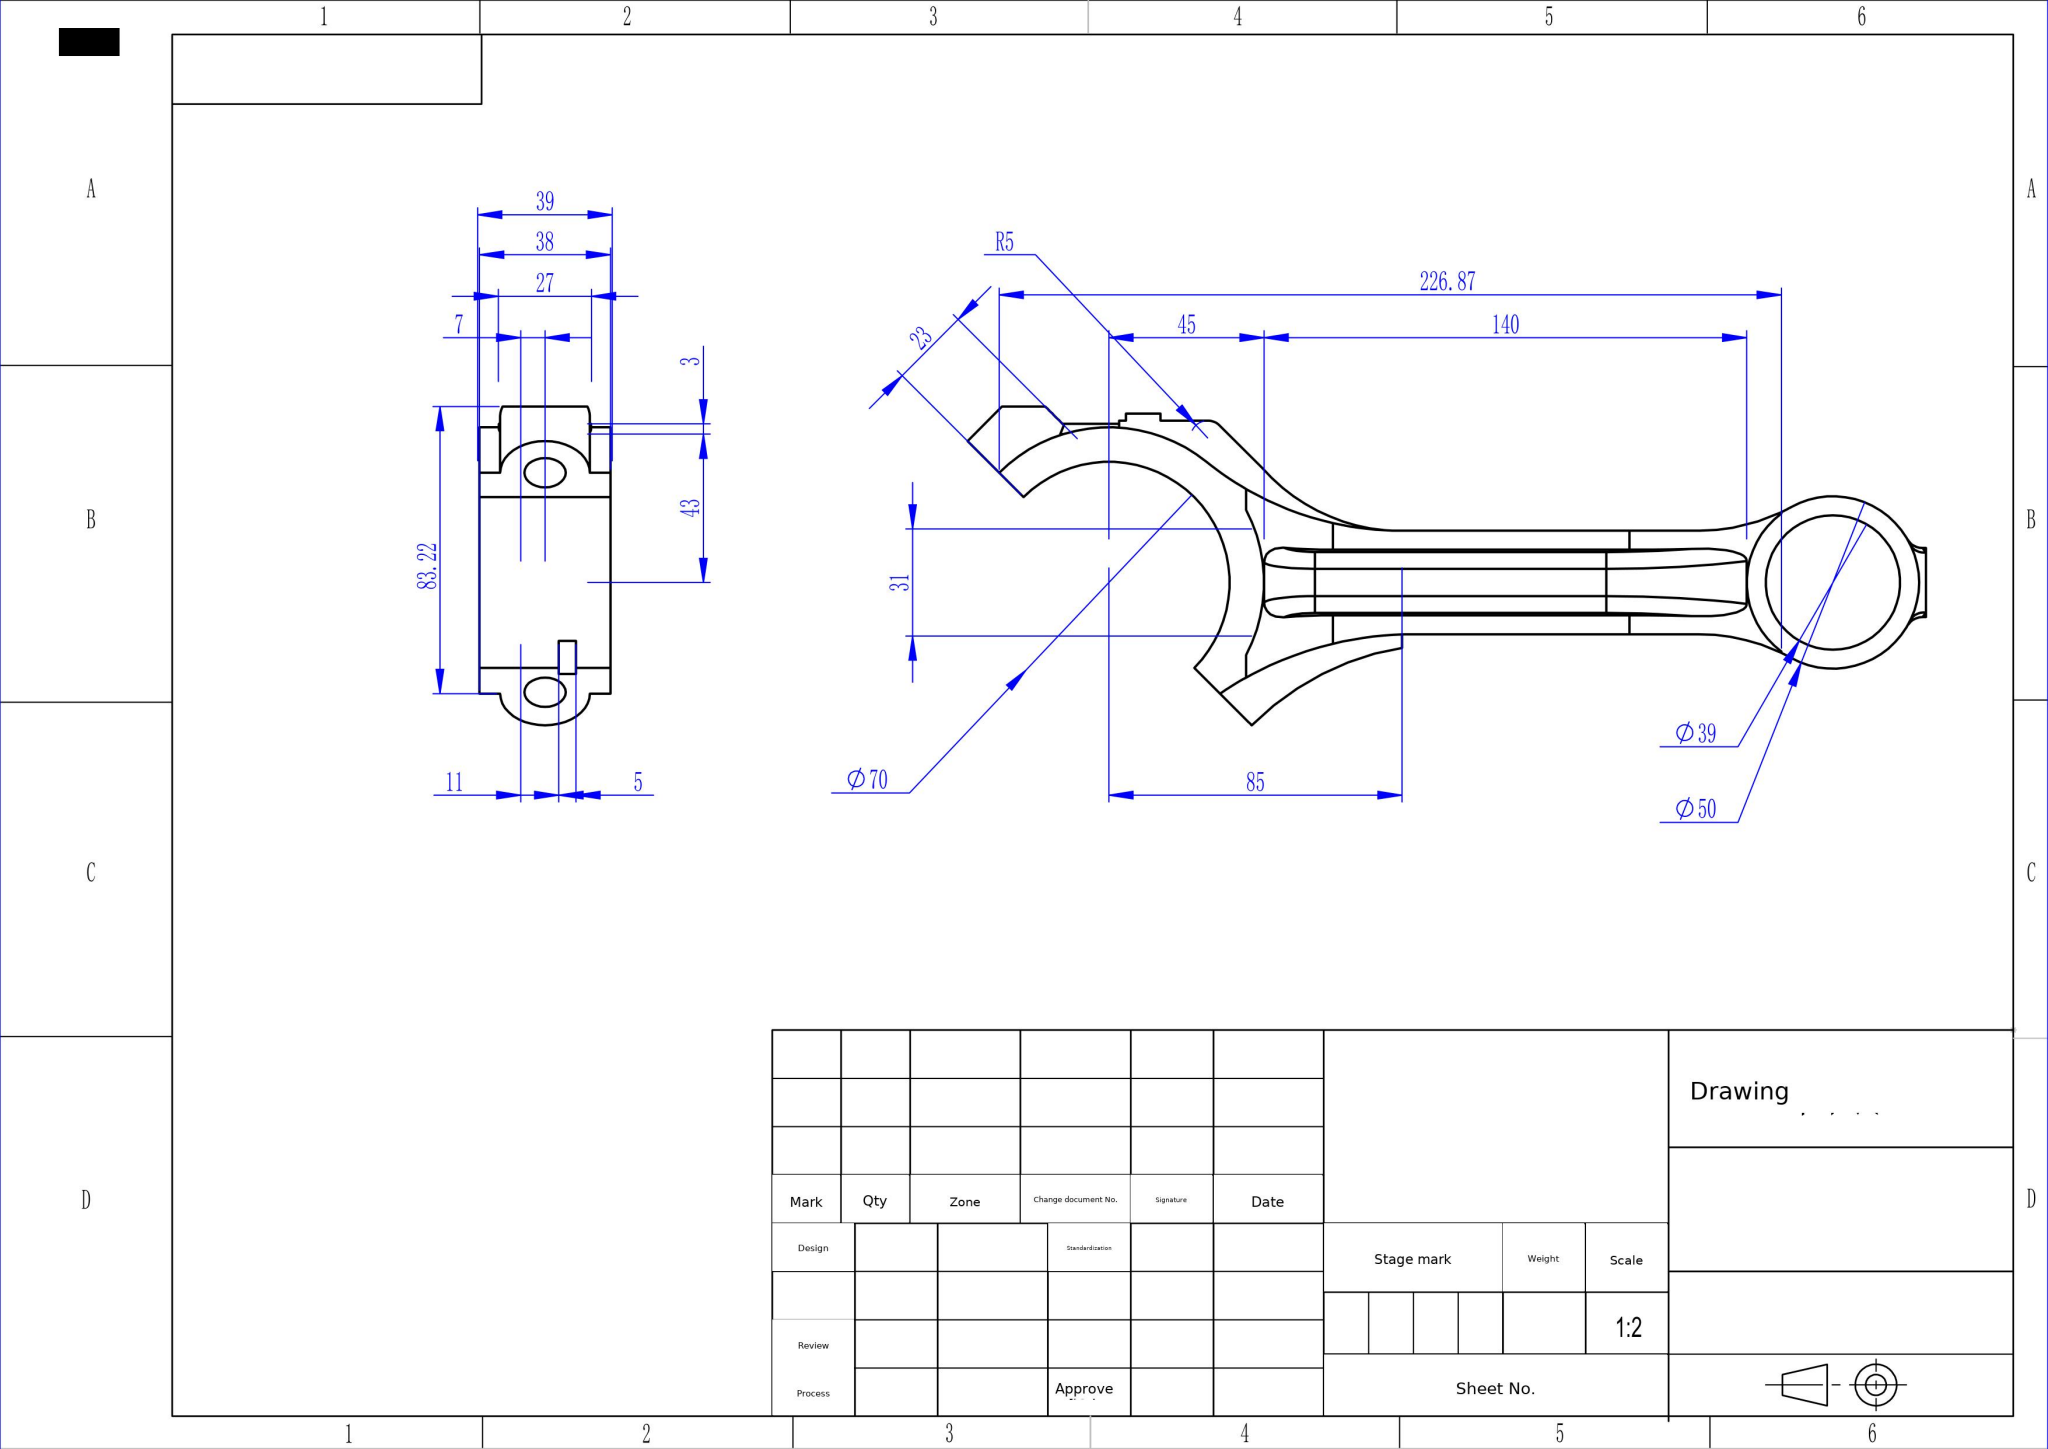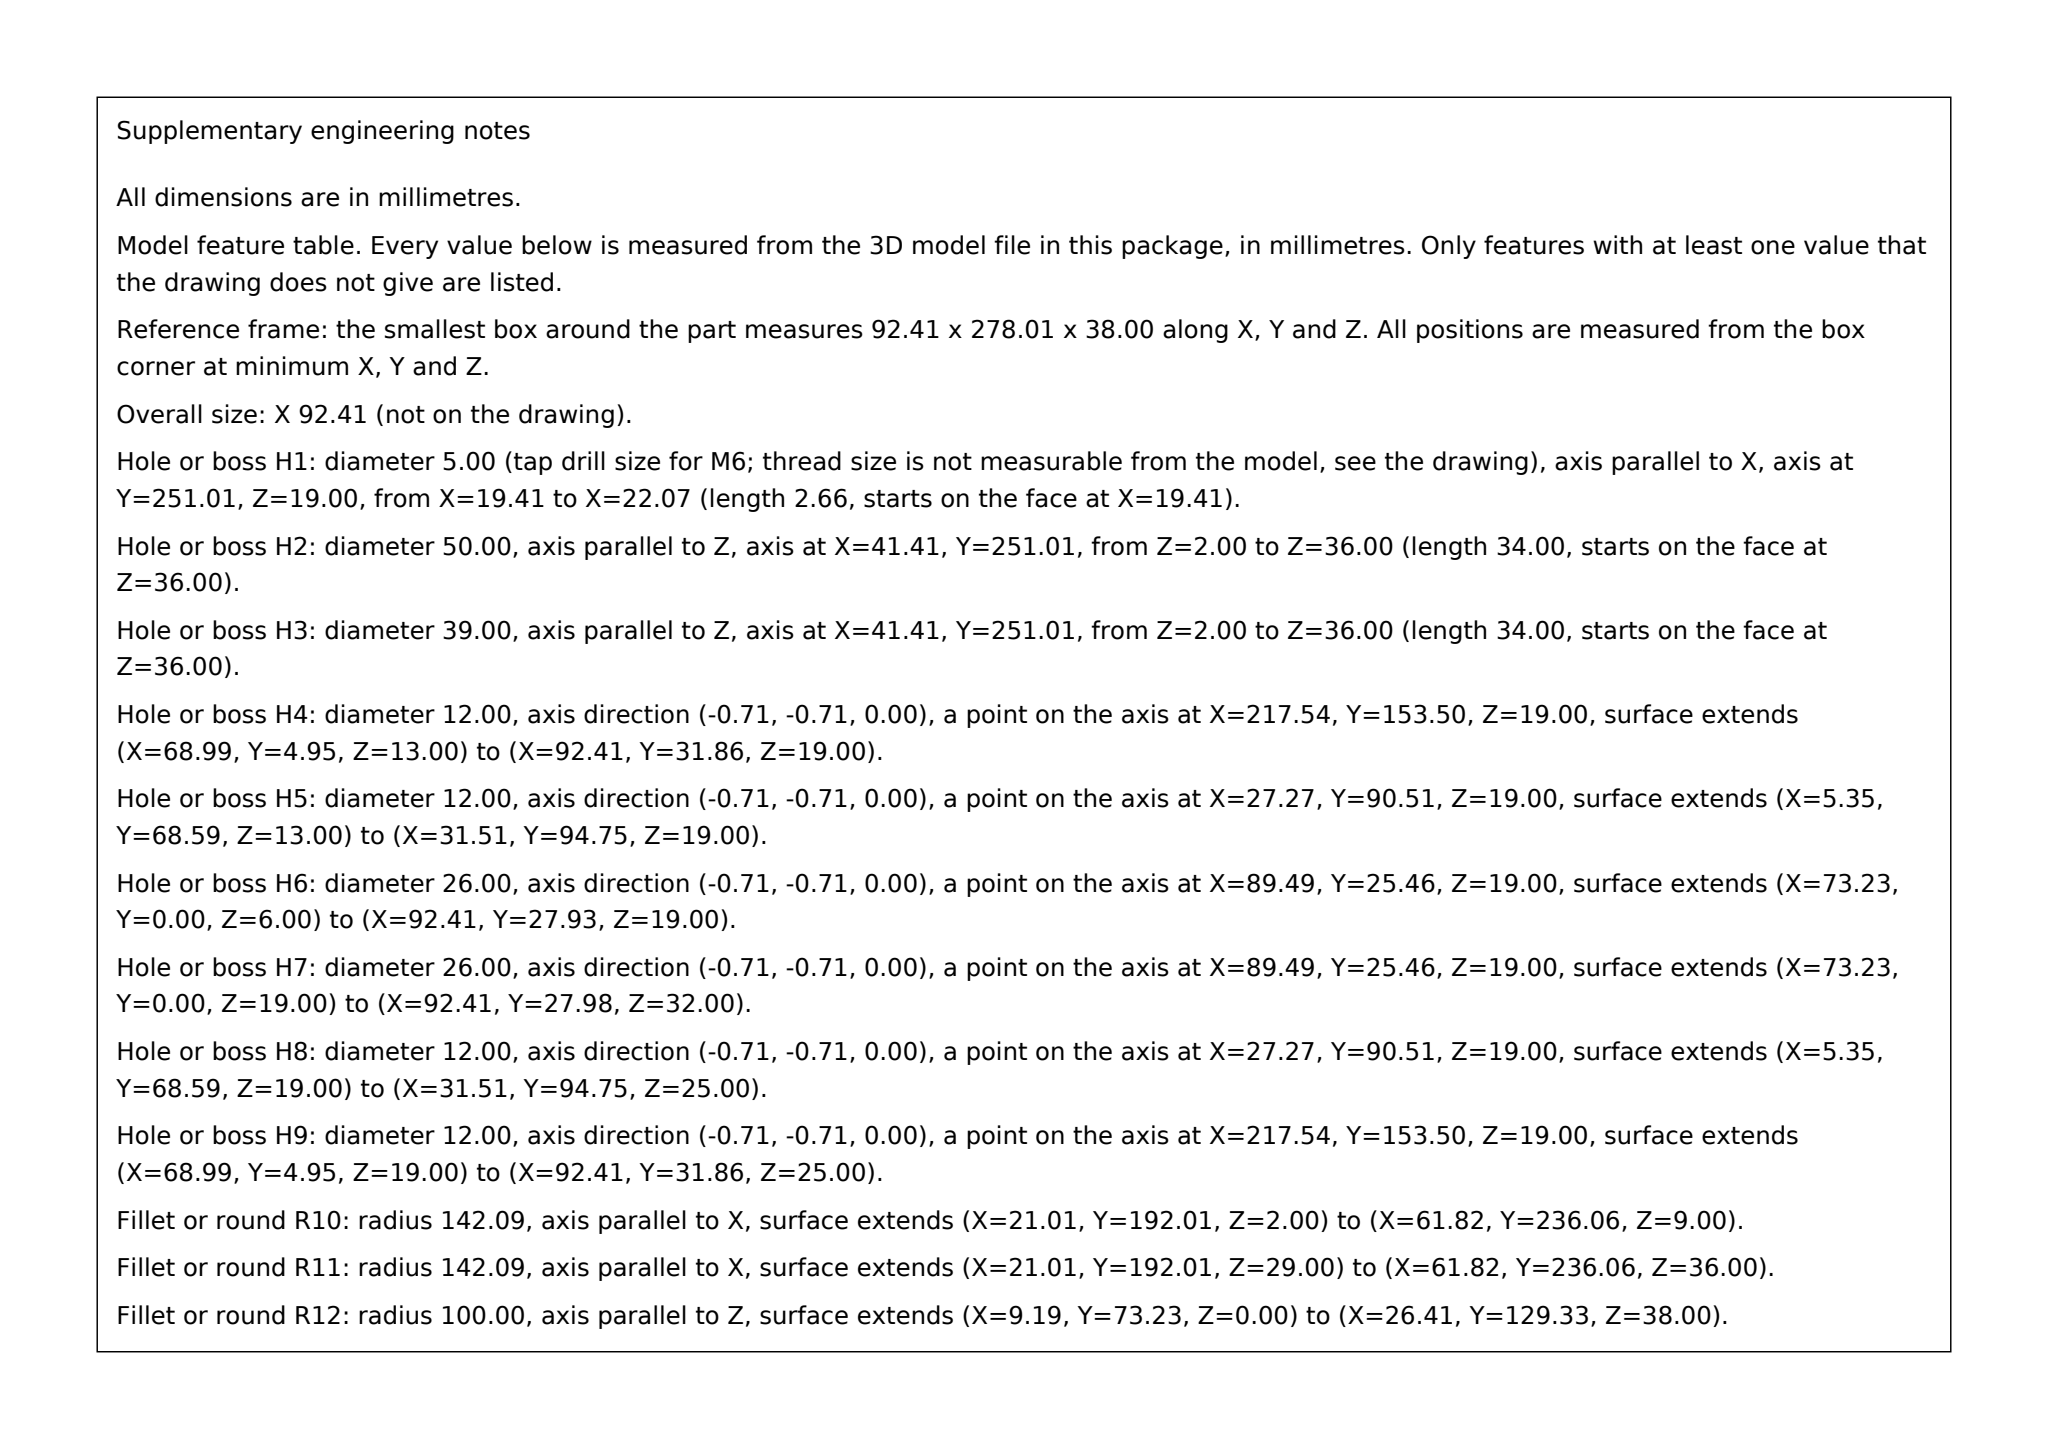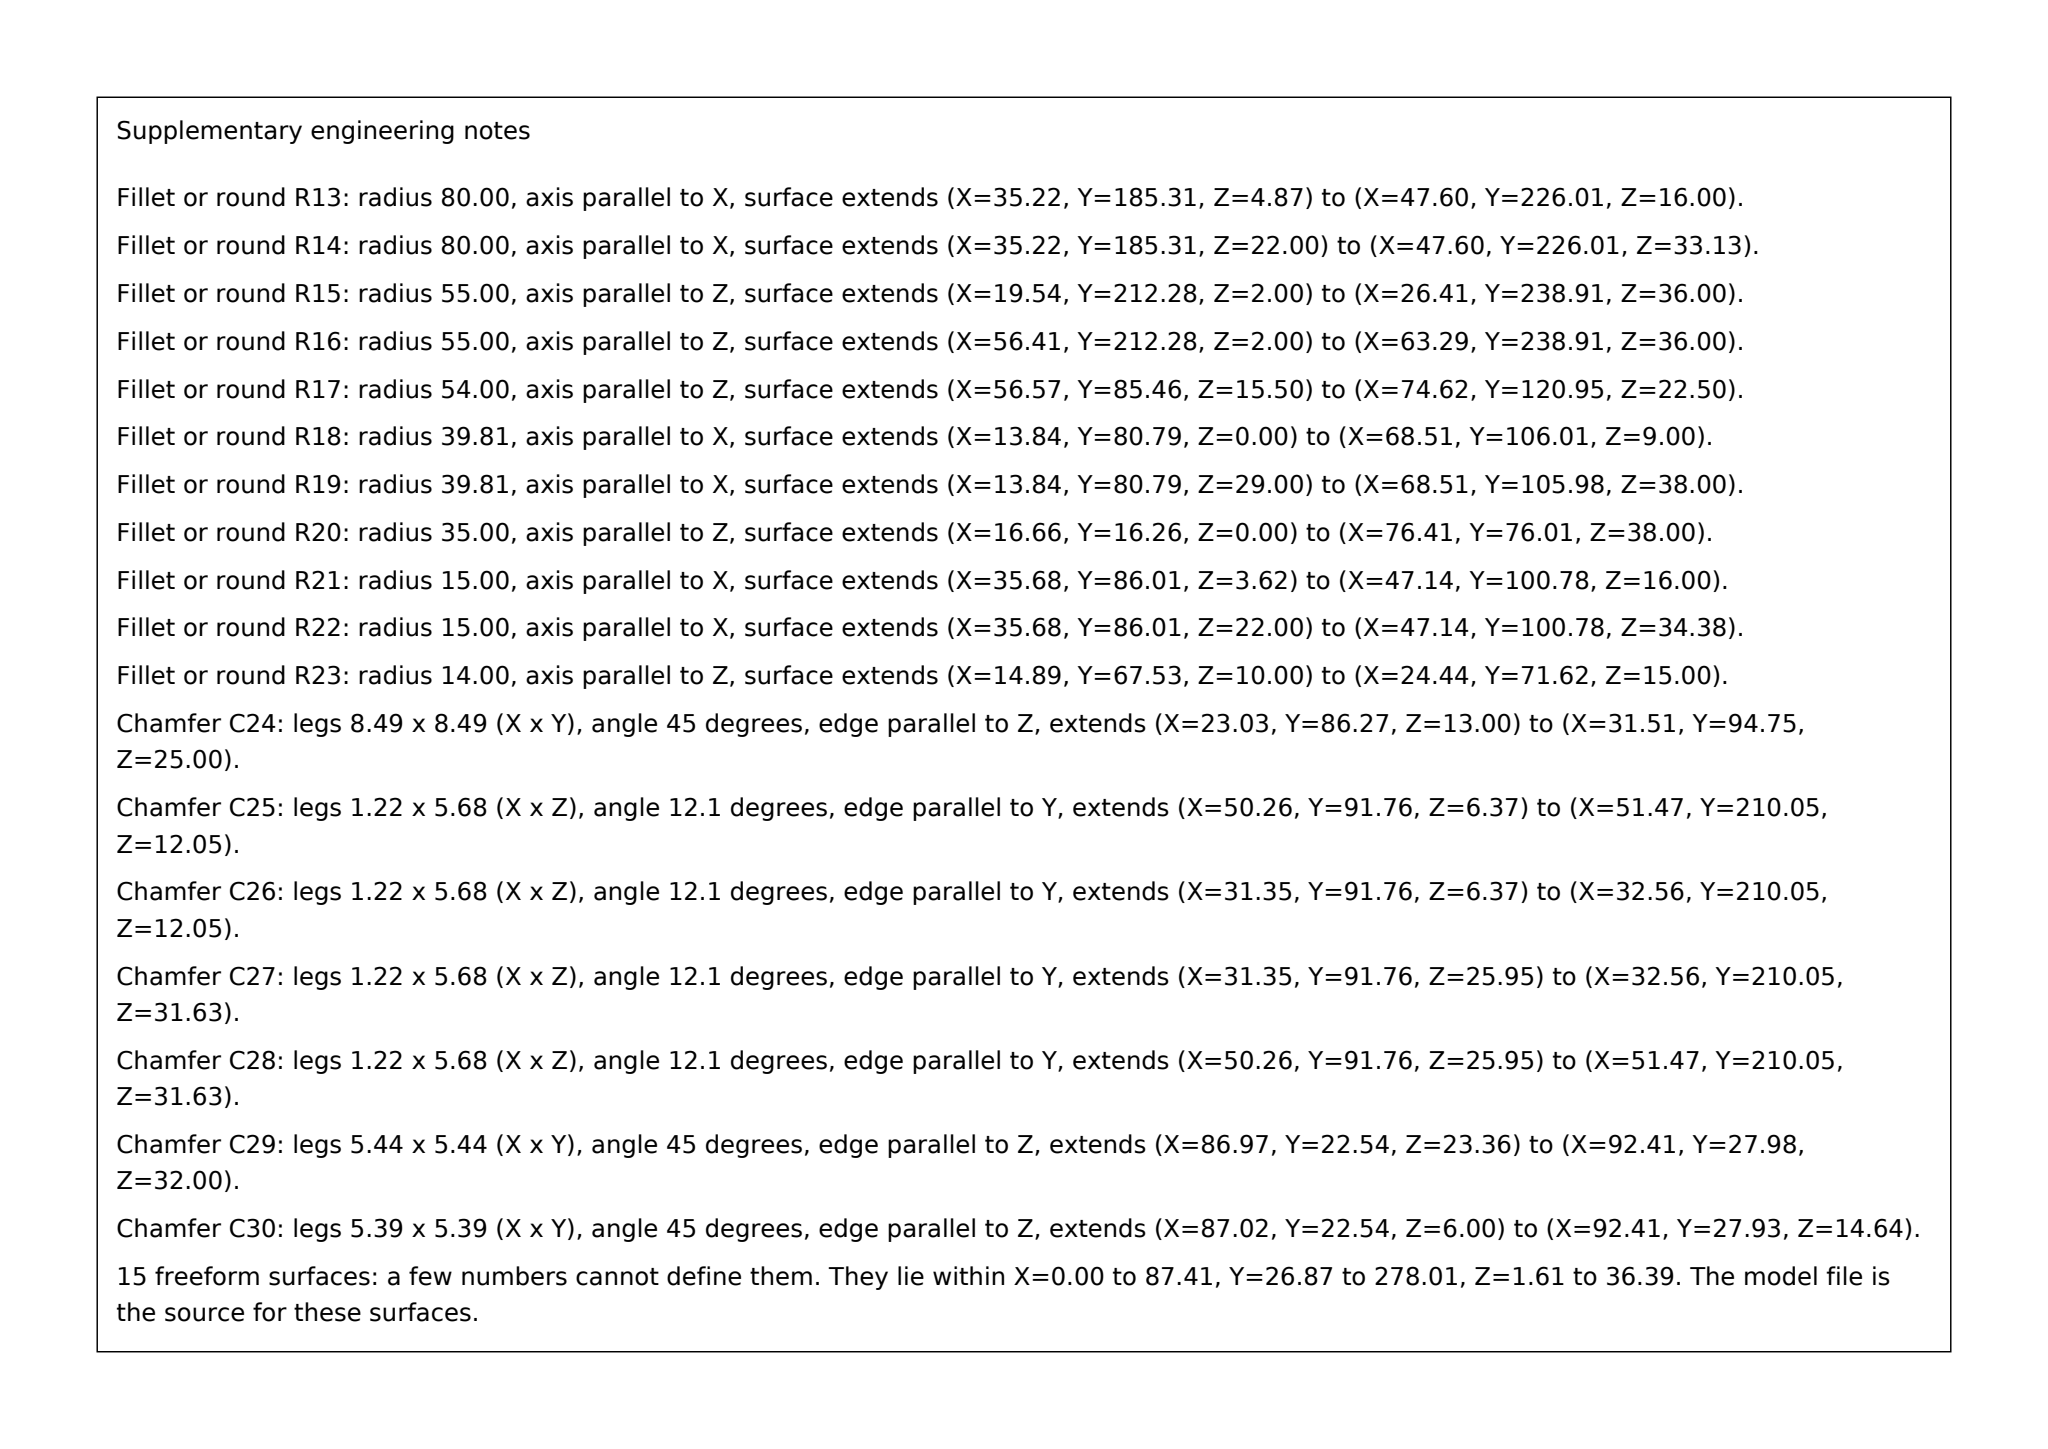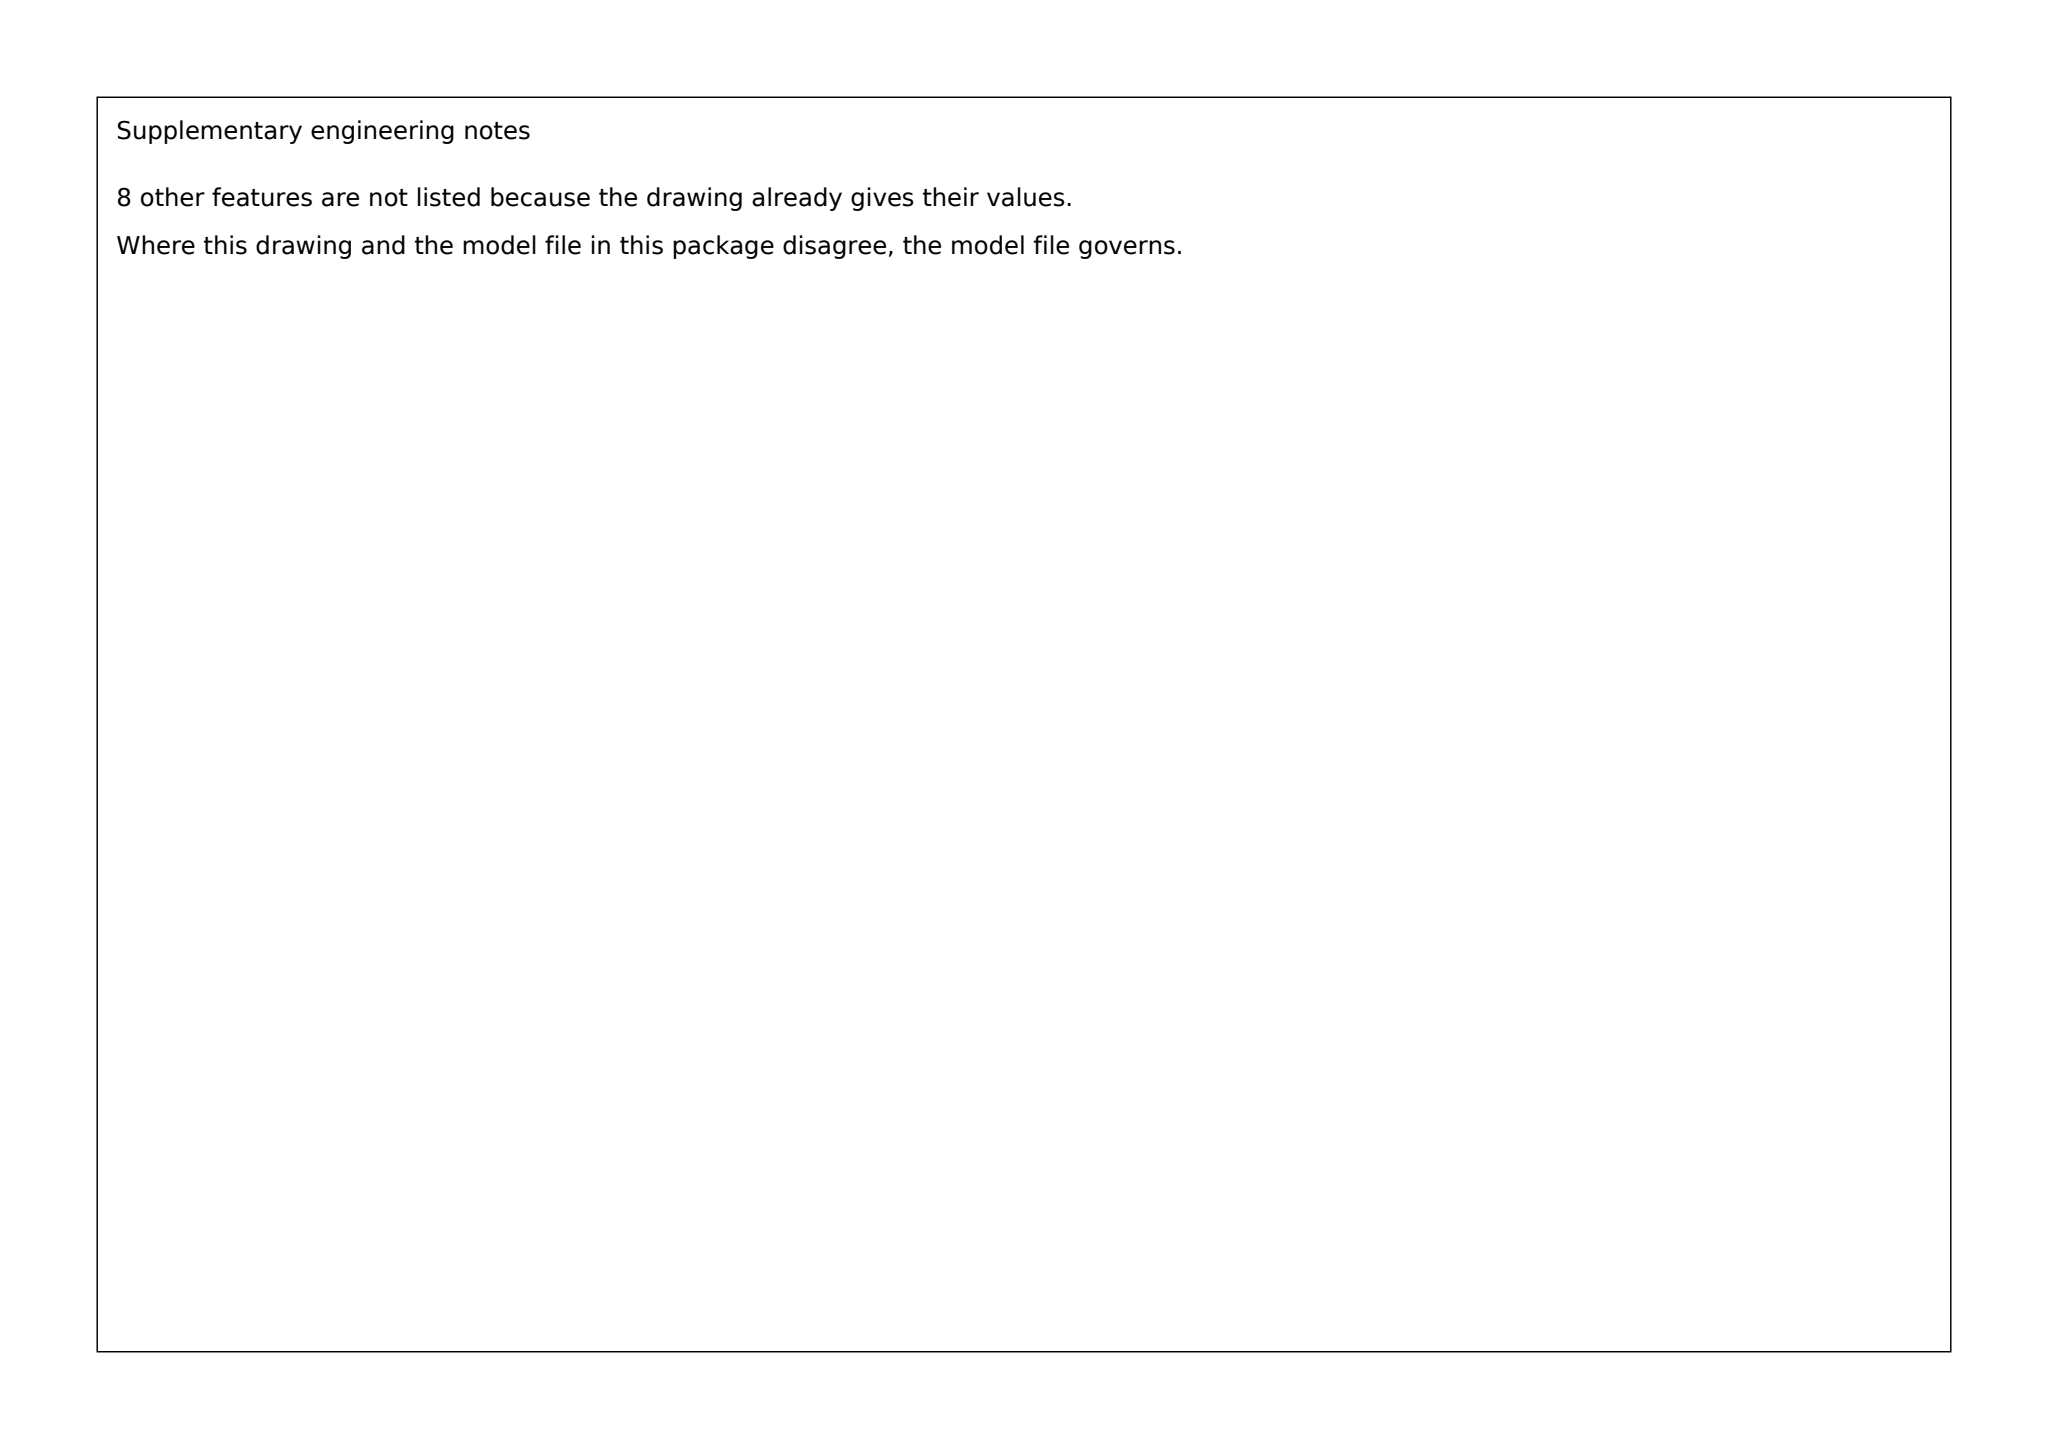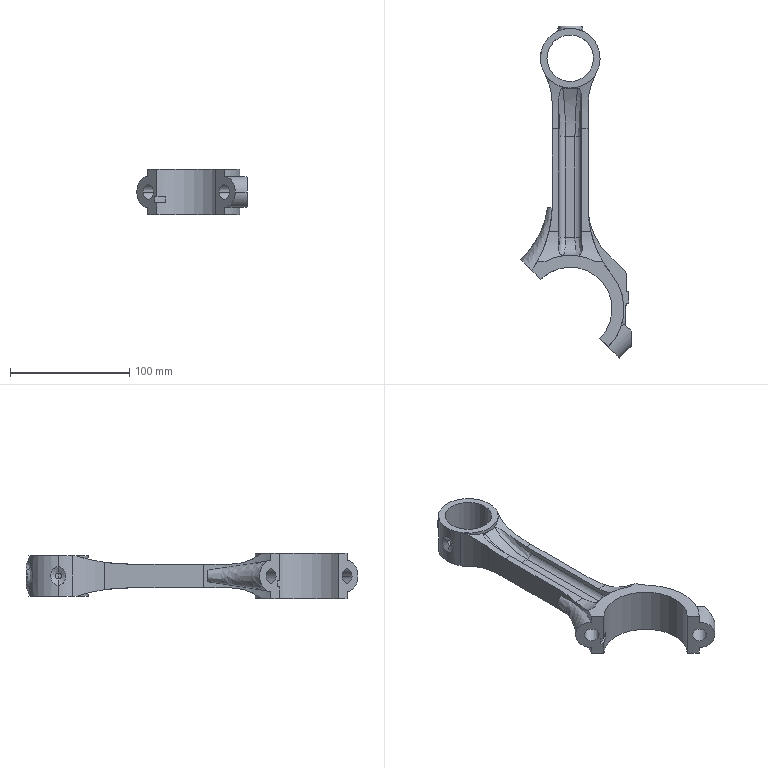Part | SolidWorks | mm | 1 solid | 102 faces | box 92.41 x 278.01 x 38 mm | volume 160940 mm3 | cylinder 46 | plane 39 | spline 15 | cone 2 | commonest cylinder face diameters 50 x5 10 x5 12 x4 90 x4 79.619 x4 284.17 x4 20 x3 5 x2